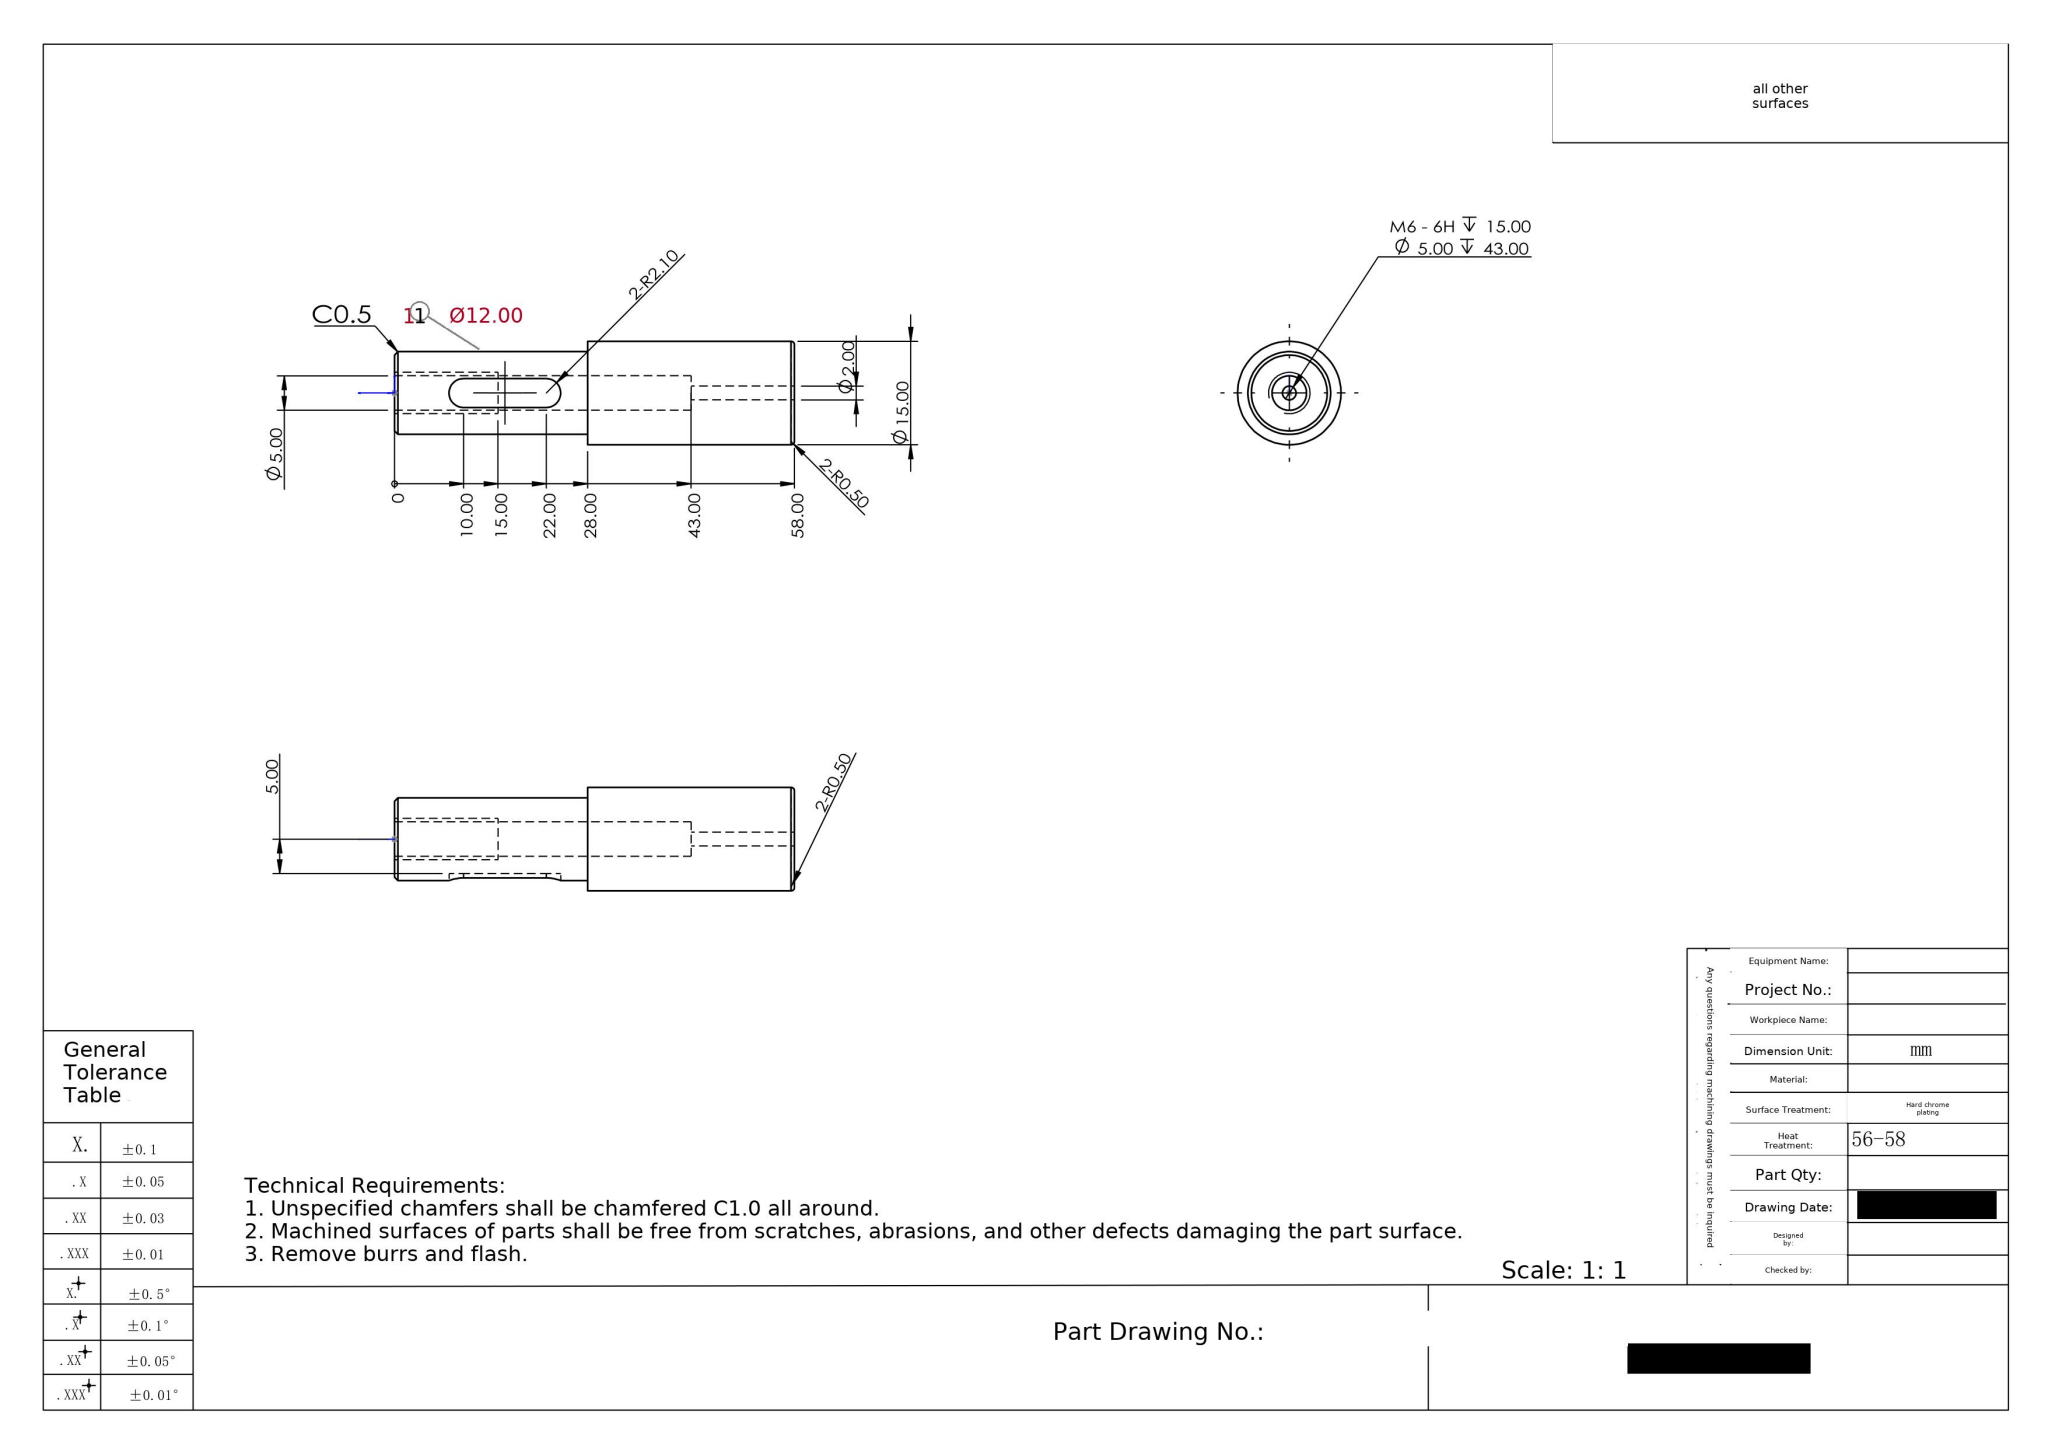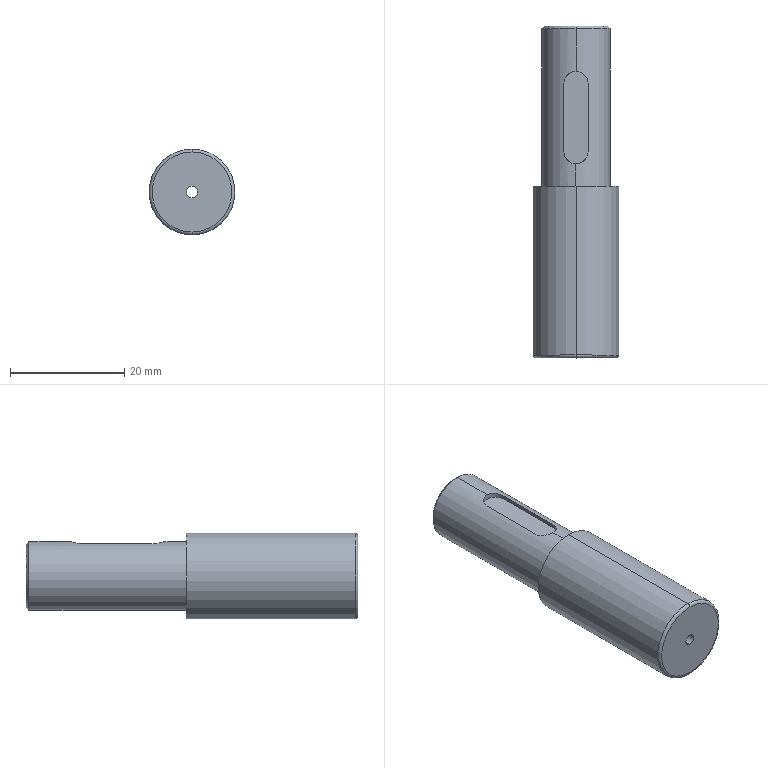Part | SolidWorks | mm | 1 solid | 21 faces | box 15 x 58 x 15 mm | volume 7513 mm3 | cylinder 10 | plane 7 | torus 2 | cone 2 | commonest cylinder face diameters 5 x2 15 x2 2 x2 12 x2 4.2 x2
build123d program:
from build123d import *

# Parameters (mm, degrees)
CUT_EXTRUDE2_START    = 5
CUT_EXTRUDE2_DEPTH    = 10
CHAMFER1_SIZE         = 0.5
M6_TAPPED_HOLE1_D     = 5
M6_TAPPED_HOLE1_DEPTH = 43
FILLET1_R             = 0.5


with BuildPart() as part:
    # Sketch1 → Revolve1 (revolve)
    with BuildSketch(Plane.XY, mode=Mode.PRIVATE) as revolve1_sk:
        Polygon((1, -58), (2.8, -58), (7.5, -58), (7.5, -47), (7.5, -28), (6, -28), (6, 0), (1, 0), align=None)
    revolve(revolve1_sk.sketch.rotate(Axis((0, 0, 0), (0, 1, 0)), 90), axis=Axis((0, 0, 0), (0, 1, 0)))

    # Sketch4 → Cut-Extrude2 (cut)
    with BuildSketch(Plane.XY.offset(CUT_EXTRUDE2_START)):
        with BuildLine():
            Line((2.1, -10), (2.1, -22))
            ThreePointArc((2.1, -22), (0, -24.1), (-2.1, -22))
            Line((-2.1, -22), (-2.1, -10))
            ThreePointArc((-2.1, -10), (0, -7.9), (2.1, -10))
        make_face()
    extrude(amount=CUT_EXTRUDE2_DEPTH, mode=Mode.SUBTRACT)

    # Chamfer1
    chamfer1_edges = [part.edges().sort_by_distance(p)[0] for p in [
        (0, 0, 6),
    ]]
    chamfer(chamfer1_edges, length=CHAMFER1_SIZE)

    # M6 Tapped Hole1
    with Locations(Plane(origin=(0, 0, 0), x_dir=(1, 0, 0), z_dir=(0, 1, 0))):
        with Locations((0, 0)):
            Hole(M6_TAPPED_HOLE1_D / 2, depth=M6_TAPPED_HOLE1_DEPTH)

    # Sketch7_2 → Cut-Revolve1 (revolve, cut)
    with BuildSketch(Plane.XY, mode=Mode.PRIVATE) as cut_revolve1_sk:
        Polygon((1, -50), (4, -50), (4, -55), (7.5, -55), (7.5, -58), (1, -58), align=None)
    revolve(cut_revolve1_sk.sketch.rotate(Axis((0, -60.339, 0), (0, 1, 0)), 90), axis=Axis((0, -60.339, 0), (0, 1, 0)), mode=Mode.SUBTRACT)

    # Sketch7_2 2 → Revolve2 (revolve)
    with BuildSketch(Plane.XY, mode=Mode.PRIVATE) as revolve2_sk:
        Polygon((1, -50), (4, -50), (4, -55), (7.5, -55), (7.5, -58), (1, -58), align=None)
    revolve(revolve2_sk.sketch.rotate(Axis((0, -60.339, 0), (0, 1, 0)), 90), axis=Axis((0, -60.339, 0), (0, 1, 0)))

    # Fillet1
    fillet1_edges = [part.edges().sort_by_distance(p)[0] for p in [
        (0, -58, 7.5),
    ]]
    fillet(fillet1_edges, radius=FILLET1_R)


solid = part.part